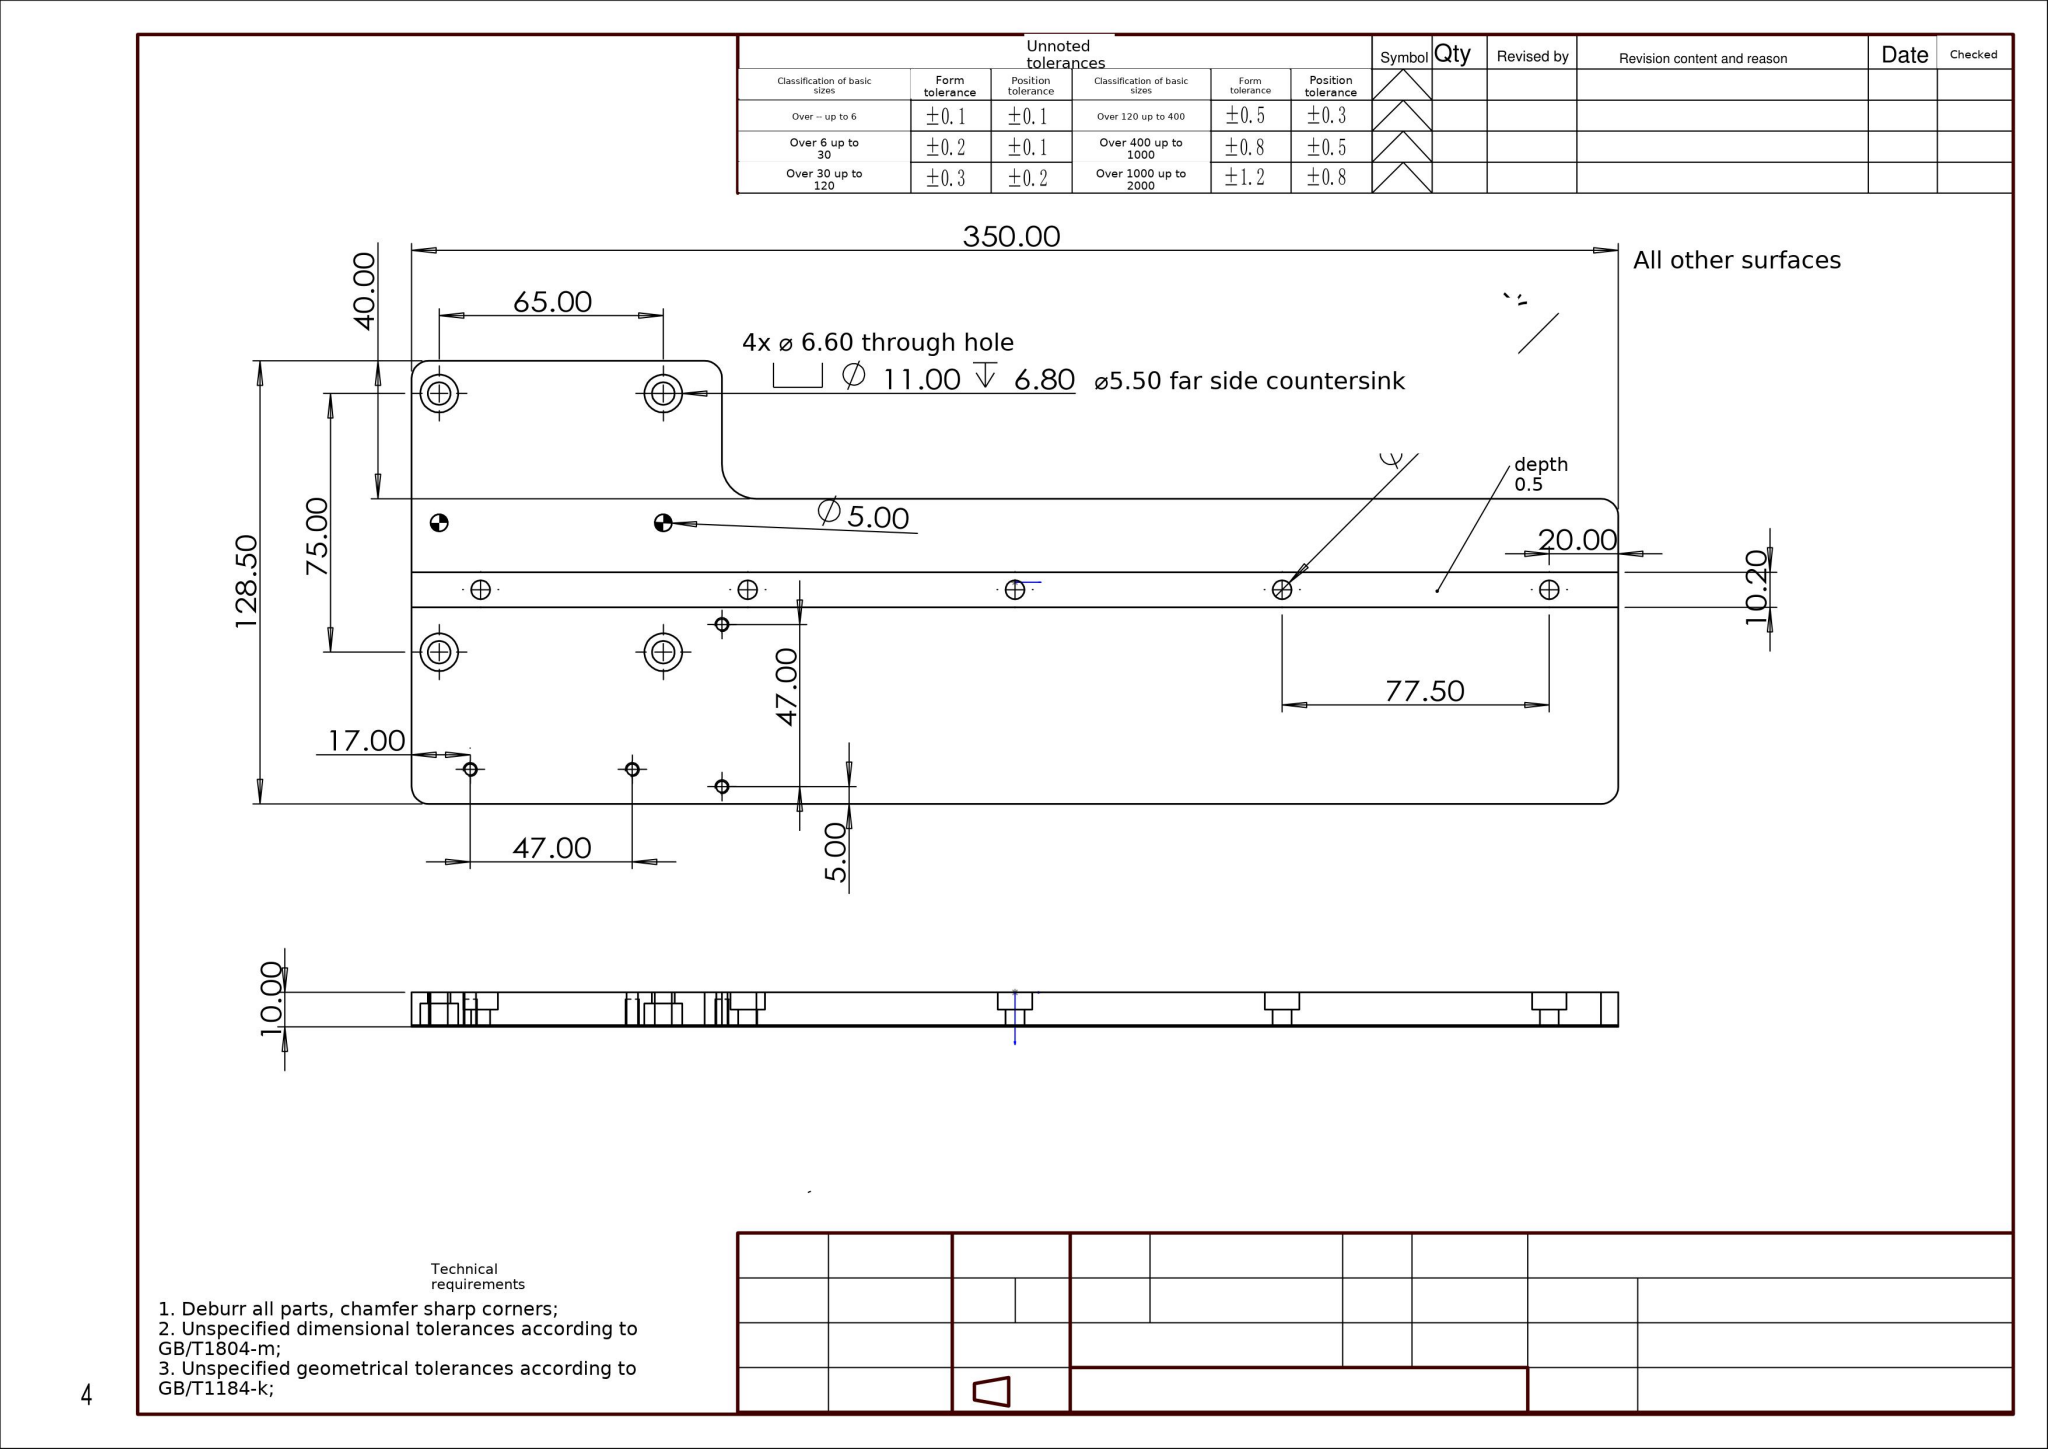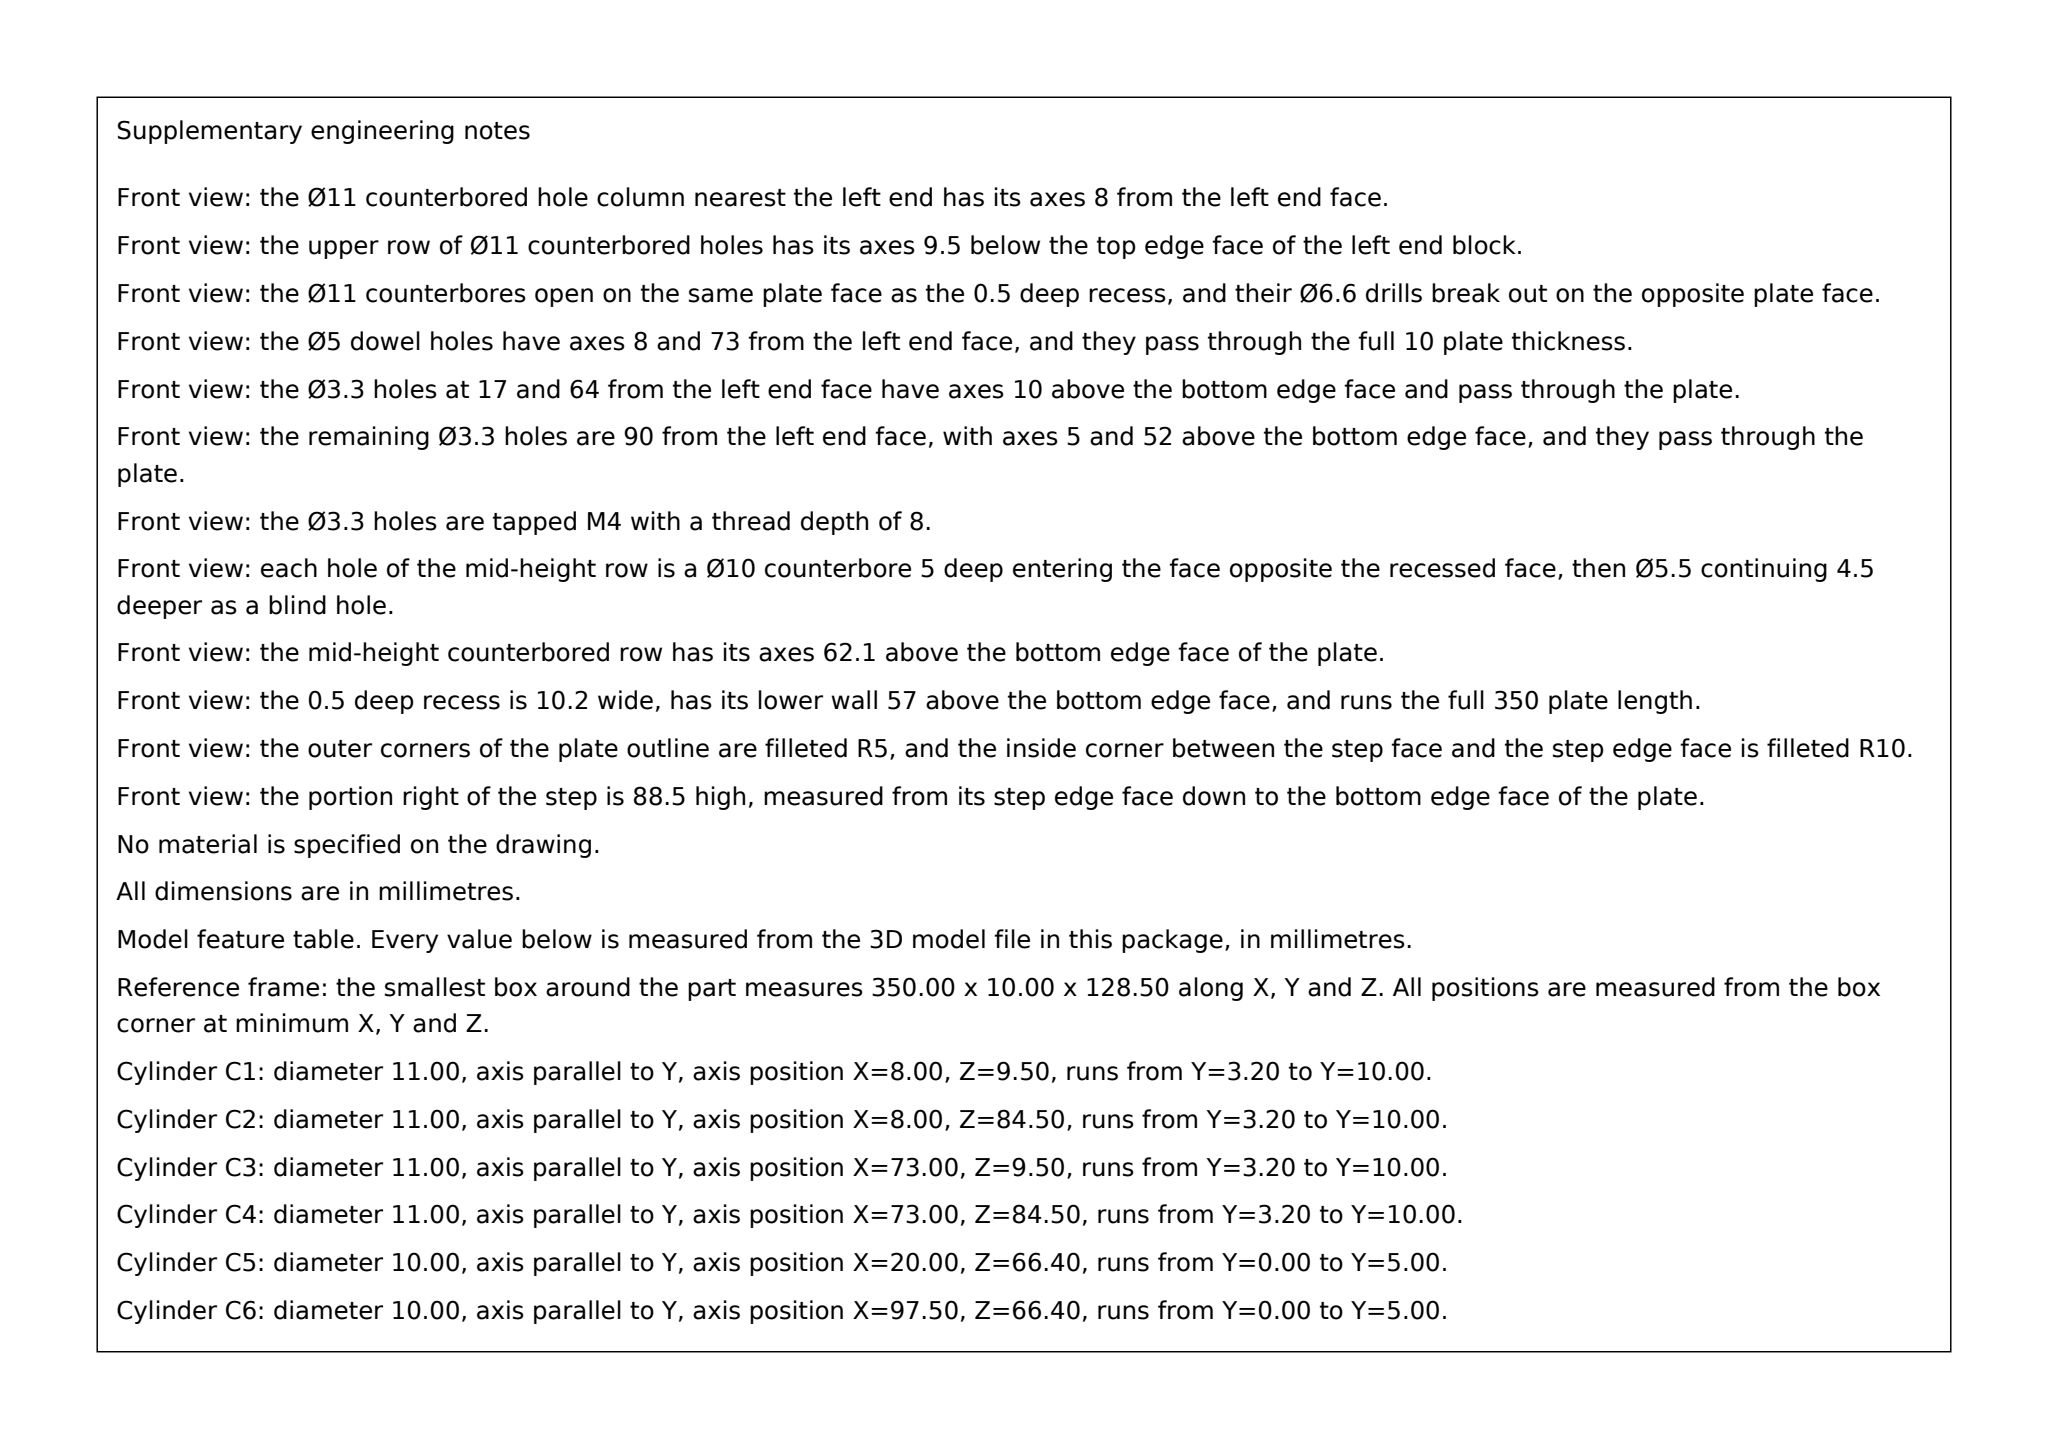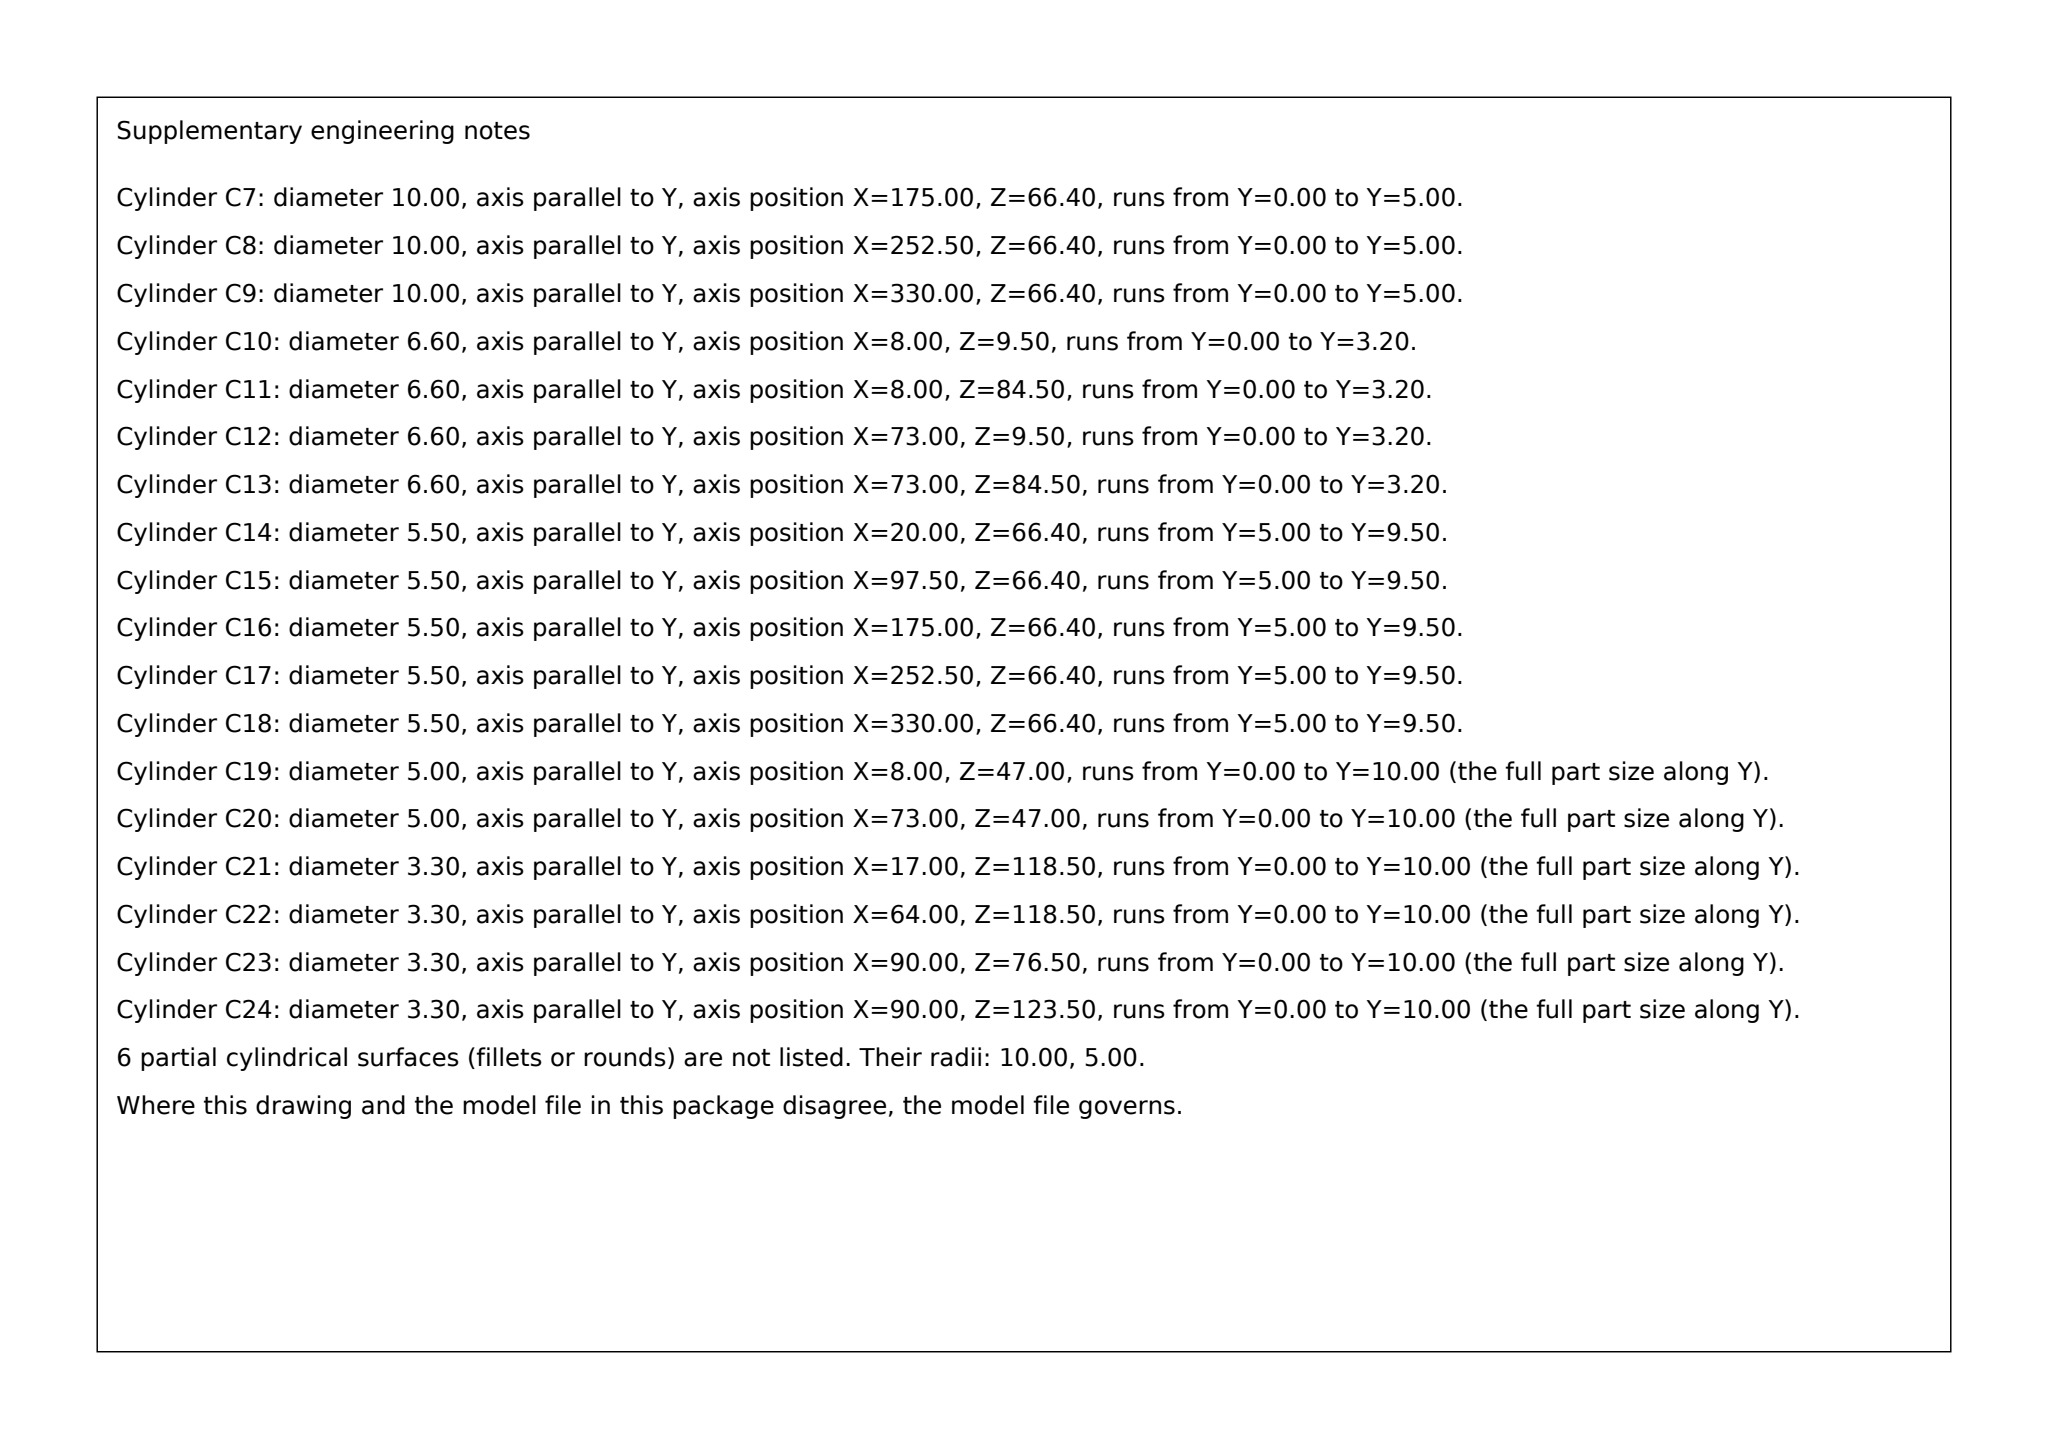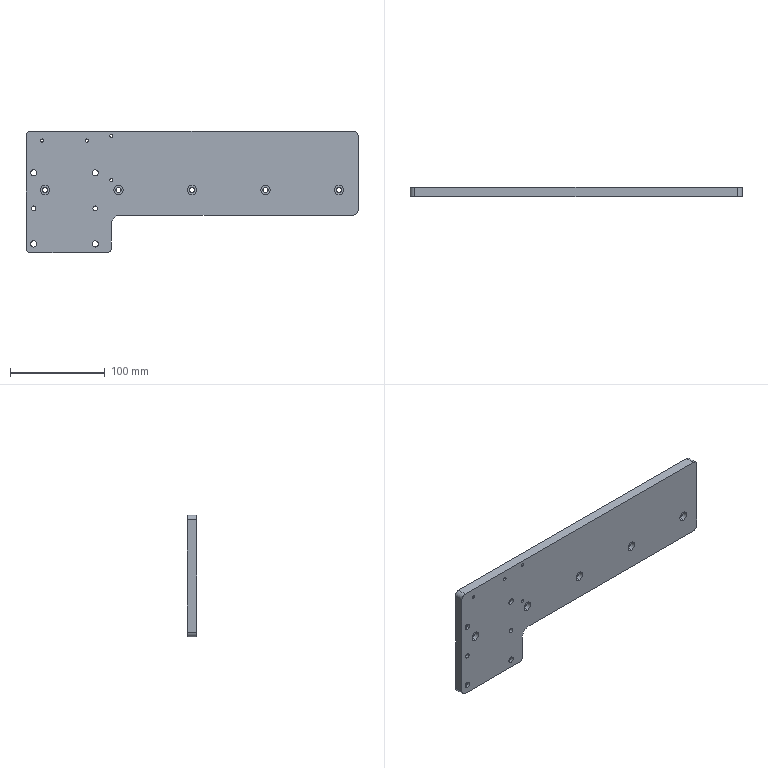Part | SolidWorks | mm | 1 solid | 75 faces | box 350 x 10 x 128.5 mm | volume 337656 mm3 | cylinder 54 | plane 21 | commonest cylinder face diameters 10 x15 5.5 x10 3.3 x8 11 x8 6.6 x8 5 x4 20 x1
Drawing notes:
4X Ø3.30 THRU (through 10.0 thk plate). | from the solid: cylinders dia 3.3, axis y, length 10.0 = full bbox Y thickness 10.0
Two Ø3.30 holes located Z=118.50 from bottom edge (10.00 from top edge), at X=17.00 and X=64.00 from left edge. | from the solid: cylinders [3.3,y,(17.0,null,118.5)] and [3.3,y,(64.0,null,118.5)]
Two Ø3.30 holes located X=90.00 from left edge, at Z=76.50 and Z=123.50 from bottom edge. | from the solid: cylinders [3.3,y,(90.0,null,76.5)] and [3.3,y,(90.0,null,123.5)]
4X Ø6.60 THRU, CBORE Ø11.00 DP 6.80: pattern at X=8.00 and X=73.00 from left edge. | from the solid: cylinders 6.6/11.0 at x=8.0 and x=73.0; 11.0 length 6.8
4X Ø6.60/CBORE Ø11.00 pattern rows at Z=9.50 and Z=84.50 from bottom edge. | from the solid: cylinders 6.6 and 11.0 at z=9.5 and z=84.5
2X Ø5.00 THRU located Z=47.00 from bottom edge, at X=8.00 and X=73.00 from left edge. | from the solid: cylinders [5.0,y,(8.0,null,47.0),10.0] and [5.0,y,(73.0,null,47.0),10.0]
Raised step/tab face at X=90.00 from left edge; step height plane at Z=40.00 from bottom edge. | from the solid: axis_planes [x,90.0] and [z,40.0]
5X Ø5.50 DP 4.50, CBORE Ø10.00 DP 5.00 (rail holes). | from the solid: cylinders [5.5,y,...,4.5] and [10.0,y,...,5.0] at same centers (20,66.4),(97.5,66.4),(175,66.4),(252.5,66.4),(330,66.4)
5X rail holes on centerline Z=66.40 from bottom edge; first hole X=20.00 from left edge, then 4X 77.50 equally spaced to X=330.00. | from the solid: cylinders 5.5 at x=20.0, 97.5, 175.0, 252.5, 330.0, all z=66.4
10.20 wide raised band bounded by Z=61.30 and Z=71.50 from bottom edge. | from the solid: axis_planes [z,61.3] and [z,71.5] (71.5-61.3=10.2)
Unspecified outer corner radii R5.00: centers at X5/Z5, X5/Z123.5, X85/Z5, X345/Z45, X345/Z123.5. | from the solid: full-depth Ø10.0 cylinders (length 10.0) at (5,5),(5,123.5),(85,5),(345,45),(345,123.5)
R10.00 inside fillet at step corner, center X=100.00, Z=30.00 from part min corner. | from the solid: cylinder [20.0,y,(100.0,null,30.0),10.0]
ALL DIMENSIONS IN MILLIMETERS. | from the solid: STEP model units mm; bbox_xyz 350.0 x 10.0 x 128.5 mm
build123d program:
from build123d import *

# Parameters (mm, degrees)
SKETCH1_W                                         = 350
SKETCH1_H                                         = 128.5
BOSS_EXTRUDE1_DEPTH                               = 10
SKETCH2_W                                         = 260
SKETCH2_H                                         = 40
CUT_EXTRUDE1_DEPTH                                = 10
HOLE_SIZE_ACCORDING_TO_TYPE_0_OF_HEXA_D           = 6.6
HOLE_SIZE_ACCORDING_TO_TYPE_0_OF_HEXA_CBORE_D     = 11
HOLE_SIZE_ACCORDING_TO_TYPE_0_OF_HEXA_CBORE_DEPTH = 6.8
SIZE_MM_DOWEL_PIN_HOLE_1_D                        = 5
SKETCH7_W                                         = 350
SKETCH7_H                                         = 10.2
CUT_EXTRUDE2_DEPTH                                = 0.5
HOLE_SIZE_ACCORDING_TO_TYPE_0_OF_2_D              = 5.5
HOLE_SIZE_ACCORDING_TO_TYPE_0_OF_2_DEPTH          = 15
HOLE_SIZE_ACCORDING_TO_TYPE_0_OF_2_CBORE_D        = 10
HOLE_SIZE_ACCORDING_TO_TYPE_0_OF_2_CBORE_DEPTH    = 5
HOLE_SIZE_ACCORDING_TO_TYPE_0_OF_2_TIP            = 1.652
M4_TAPPED_HOLE1_D                                 = 3.3
M4_TAPPED_HOLE1_DEPTH                             = 12.4
M4_TAPPED_HOLE1_TIP                               = 0.9914
FILLET1_R                                         = 10
FILLET2_R                                         = 5
M4X0_7_TAPPED_HOLE1_D                             = 3.3
M4X0_7_TAPPED_HOLE1_DEPTH                         = 10.1
M4X0_7_TAPPED_HOLE1_TIP                           = 0.9914


with BuildPart() as part:
    # Sketch1 → Boss-Extrude1 (new body)
    with BuildSketch(Plane(origin=(0, 0, 0), x_dir=(1, 0, 0), z_dir=(0, 1, 0))):
        Rectangle(SKETCH1_W, SKETCH1_H)
    extrude(amount=BOSS_EXTRUDE1_DEPTH)

    # Sketch2 → Cut-Extrude1 (cut)
    with BuildSketch(Plane(origin=(0, 10, 0), x_dir=(1, 0, 0), z_dir=(0, 1, 0))):
        with Locations((45, 44.25)):
            Rectangle(SKETCH2_W, SKETCH2_H)
    extrude(amount=-CUT_EXTRUDE1_DEPTH, mode=Mode.SUBTRACT)

    # Hole Size _ according to_ Type 0 of Hexa (through all)
    with Locations(Plane(origin=(0, 10, 0), x_dir=(1, 0, 0), z_dir=(0, 1, 0))):
        with Locations((-167, 54.75), (-102, 54.75), (-102, -20.25), (-167, -20.25)):
            CounterBoreHole(HOLE_SIZE_ACCORDING_TO_TYPE_0_OF_HEXA_D / 2, HOLE_SIZE_ACCORDING_TO_TYPE_0_OF_HEXA_CBORE_D / 2, HOLE_SIZE_ACCORDING_TO_TYPE_0_OF_HEXA_CBORE_DEPTH)

    # Size mm Dowel Pin Hole 1 (through all)
    with Locations(Plane(origin=(0, 10, 0), x_dir=(1, 0, 0), z_dir=(0, 1, 0))):
        with Locations((-167, 17.25), (-102, 17.25)):
            Hole(SIZE_MM_DOWEL_PIN_HOLE_1_D / 2)

    # Sketch7 → Cut-Extrude2 (cut)
    with BuildSketch(Plane(origin=(0, 10, 0), x_dir=(1, 0, 0), z_dir=(0, 1, 0))):
        with Locations((0, -2.15)):
            Rectangle(SKETCH7_W, SKETCH7_H)
    extrude(amount=-CUT_EXTRUDE2_DEPTH, mode=Mode.SUBTRACT)

    # Hole Size _ according to_ Type 0 of  2
    with Locations(Plane(origin=(0, 0, 0), x_dir=(-1, 0, 0), z_dir=(0, -1, 0))):
        with Locations((155, -2.15), (-155, -2.15), (77.5, -2.15), (0, -2.15), (-77.5, -2.15)):
            CounterBoreHole(HOLE_SIZE_ACCORDING_TO_TYPE_0_OF_2_D / 2, HOLE_SIZE_ACCORDING_TO_TYPE_0_OF_2_CBORE_D / 2, HOLE_SIZE_ACCORDING_TO_TYPE_0_OF_2_CBORE_DEPTH, depth=HOLE_SIZE_ACCORDING_TO_TYPE_0_OF_2_DEPTH)
            with Locations((0, 0, -(HOLE_SIZE_ACCORDING_TO_TYPE_0_OF_2_DEPTH + HOLE_SIZE_ACCORDING_TO_TYPE_0_OF_2_TIP / 2))):  # 118° drill point
                Cone(0, HOLE_SIZE_ACCORDING_TO_TYPE_0_OF_2_D / 2, HOLE_SIZE_ACCORDING_TO_TYPE_0_OF_2_TIP, mode=Mode.SUBTRACT)

    # M4 Tapped Hole1
    with Locations(Plane(origin=(0, 10, 0), x_dir=(1, 0, 0), z_dir=(0, 1, 0))):
        with Locations((-85, -12.25), (-85, -59.25)):
            Hole(M4_TAPPED_HOLE1_D / 2, depth=M4_TAPPED_HOLE1_DEPTH)
            with Locations((0, 0, -(M4_TAPPED_HOLE1_DEPTH + M4_TAPPED_HOLE1_TIP / 2))):  # 118° drill point
                Cone(0, M4_TAPPED_HOLE1_D / 2, M4_TAPPED_HOLE1_TIP, mode=Mode.SUBTRACT)

    # Fillet1
    fillet1_edges = [part.edges().sort_by_distance(p)[0] for p in [
        (-85, 5, -24.25),
    ]]
    fillet(fillet1_edges, radius=FILLET1_R)

    # Fillet2
    fillet2_edges = [part.edges().sort_by_distance(p)[0] for p in [
        (175, 5, -24.25),
        (-85, 5, -64.25),
        (175, 5, 64.25),
        (-175, 5, 64.25),
        (-175, 5, -64.25),
    ]]
    fillet(fillet2_edges, radius=FILLET2_R)

    # M4x0.7 Tapped Hole1
    with Locations(Plane(origin=(0, 10, 0), x_dir=(1, 0, 0), z_dir=(0, 1, 0))):
        with Locations((-158, -54.25), (-111, -54.25)):
            Hole(M4X0_7_TAPPED_HOLE1_D / 2, depth=M4X0_7_TAPPED_HOLE1_DEPTH)
            with Locations((0, 0, -(M4X0_7_TAPPED_HOLE1_DEPTH + M4X0_7_TAPPED_HOLE1_TIP / 2))):  # 118° drill point
                Cone(0, M4X0_7_TAPPED_HOLE1_D / 2, M4X0_7_TAPPED_HOLE1_TIP, mode=Mode.SUBTRACT)


solid = part.part